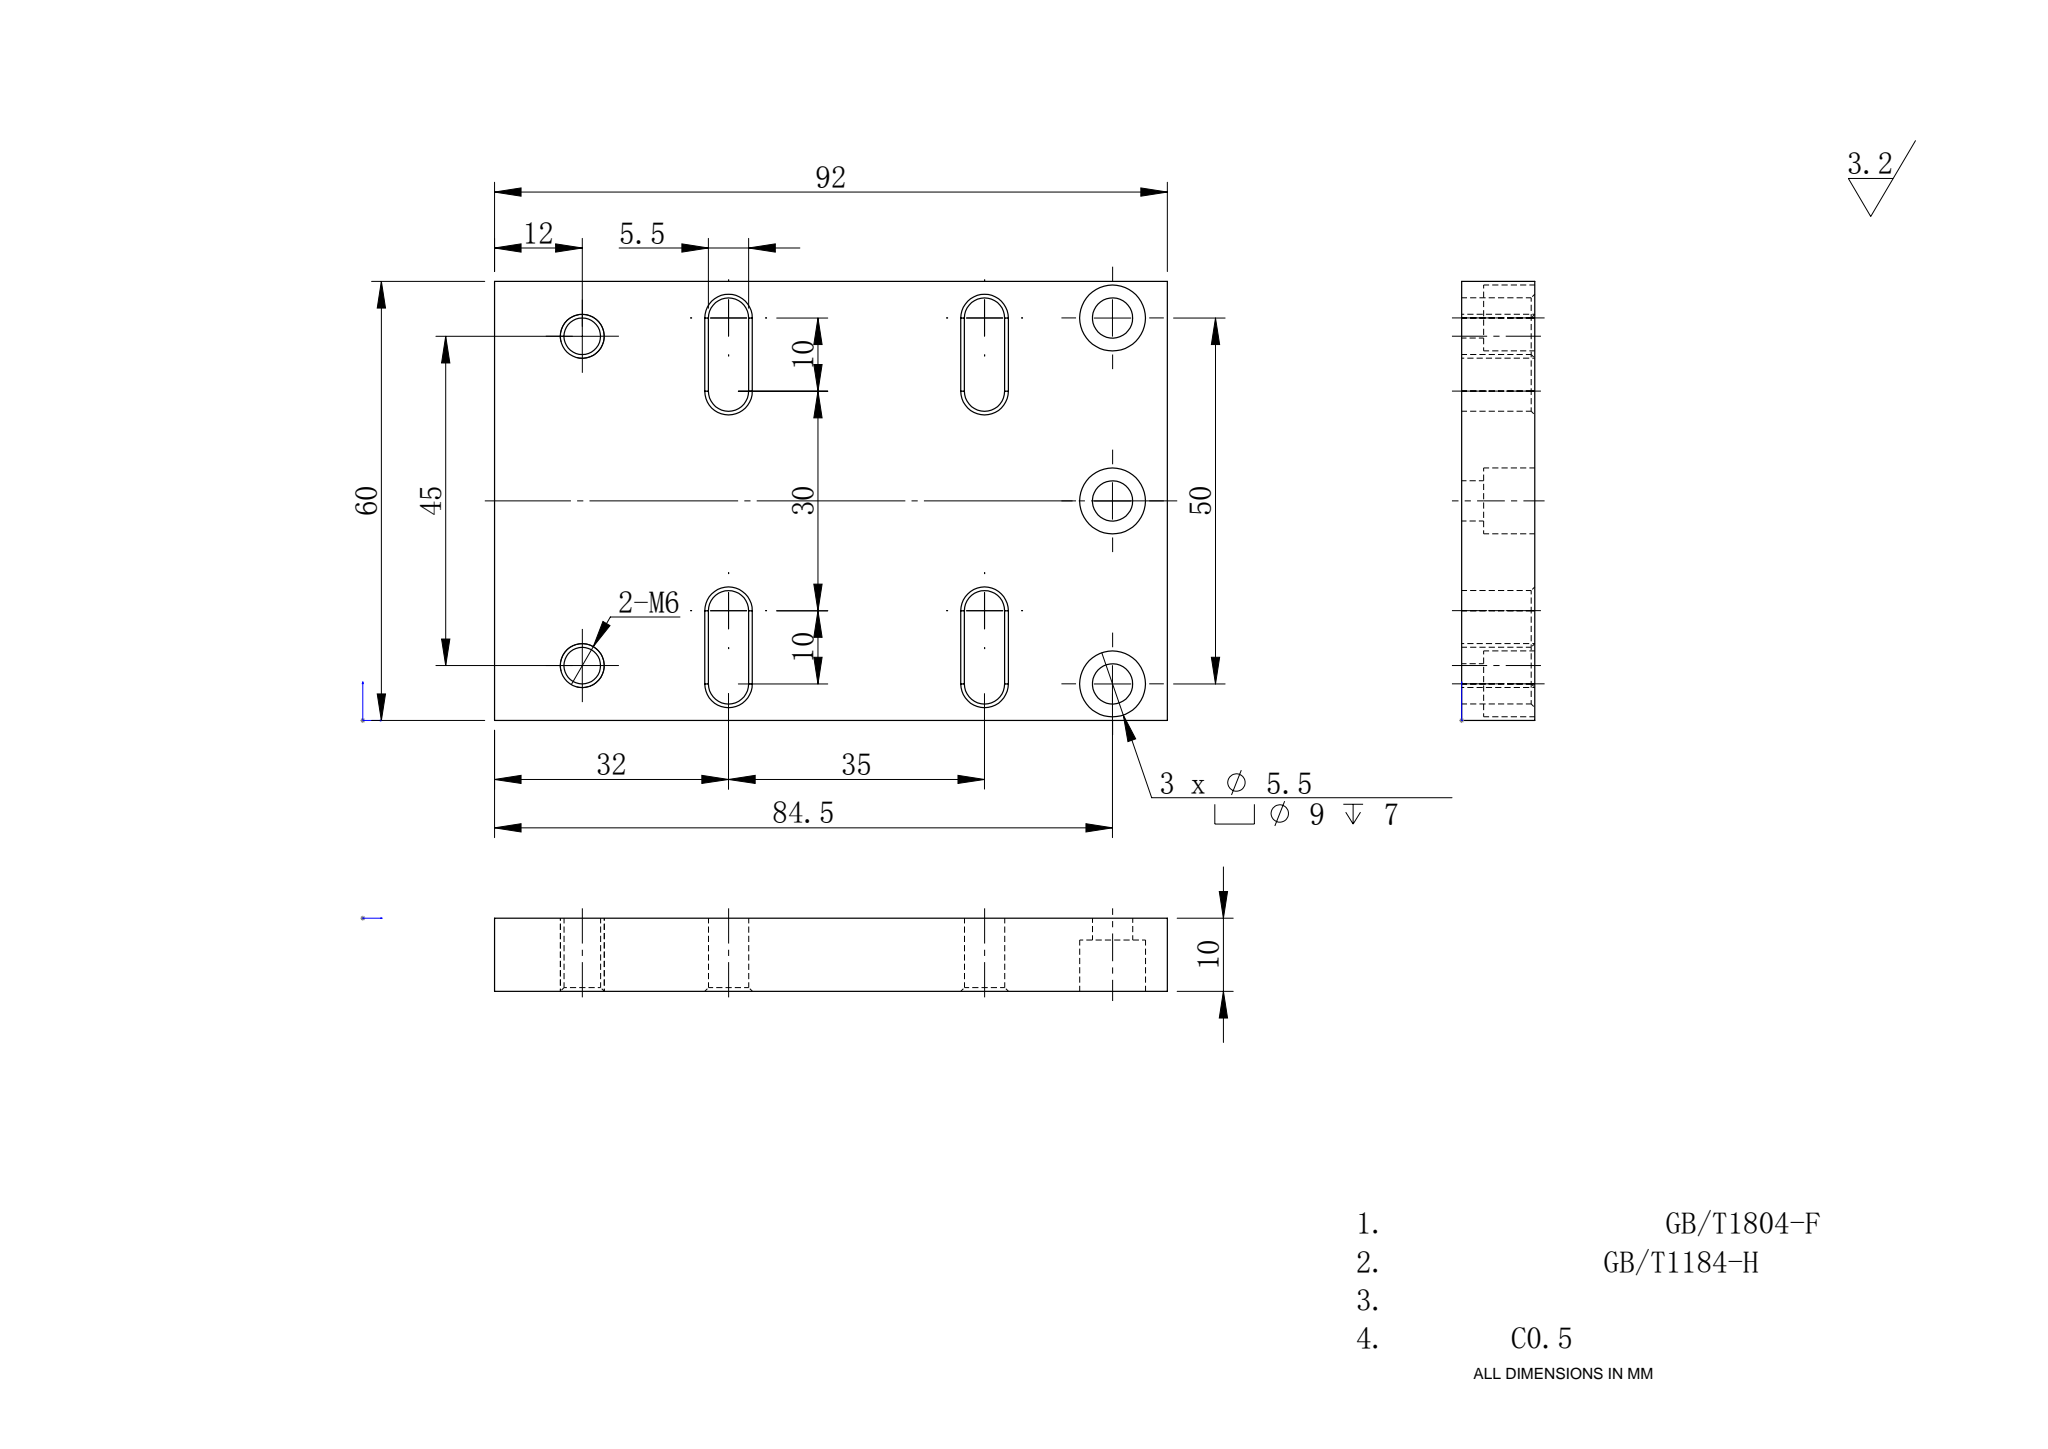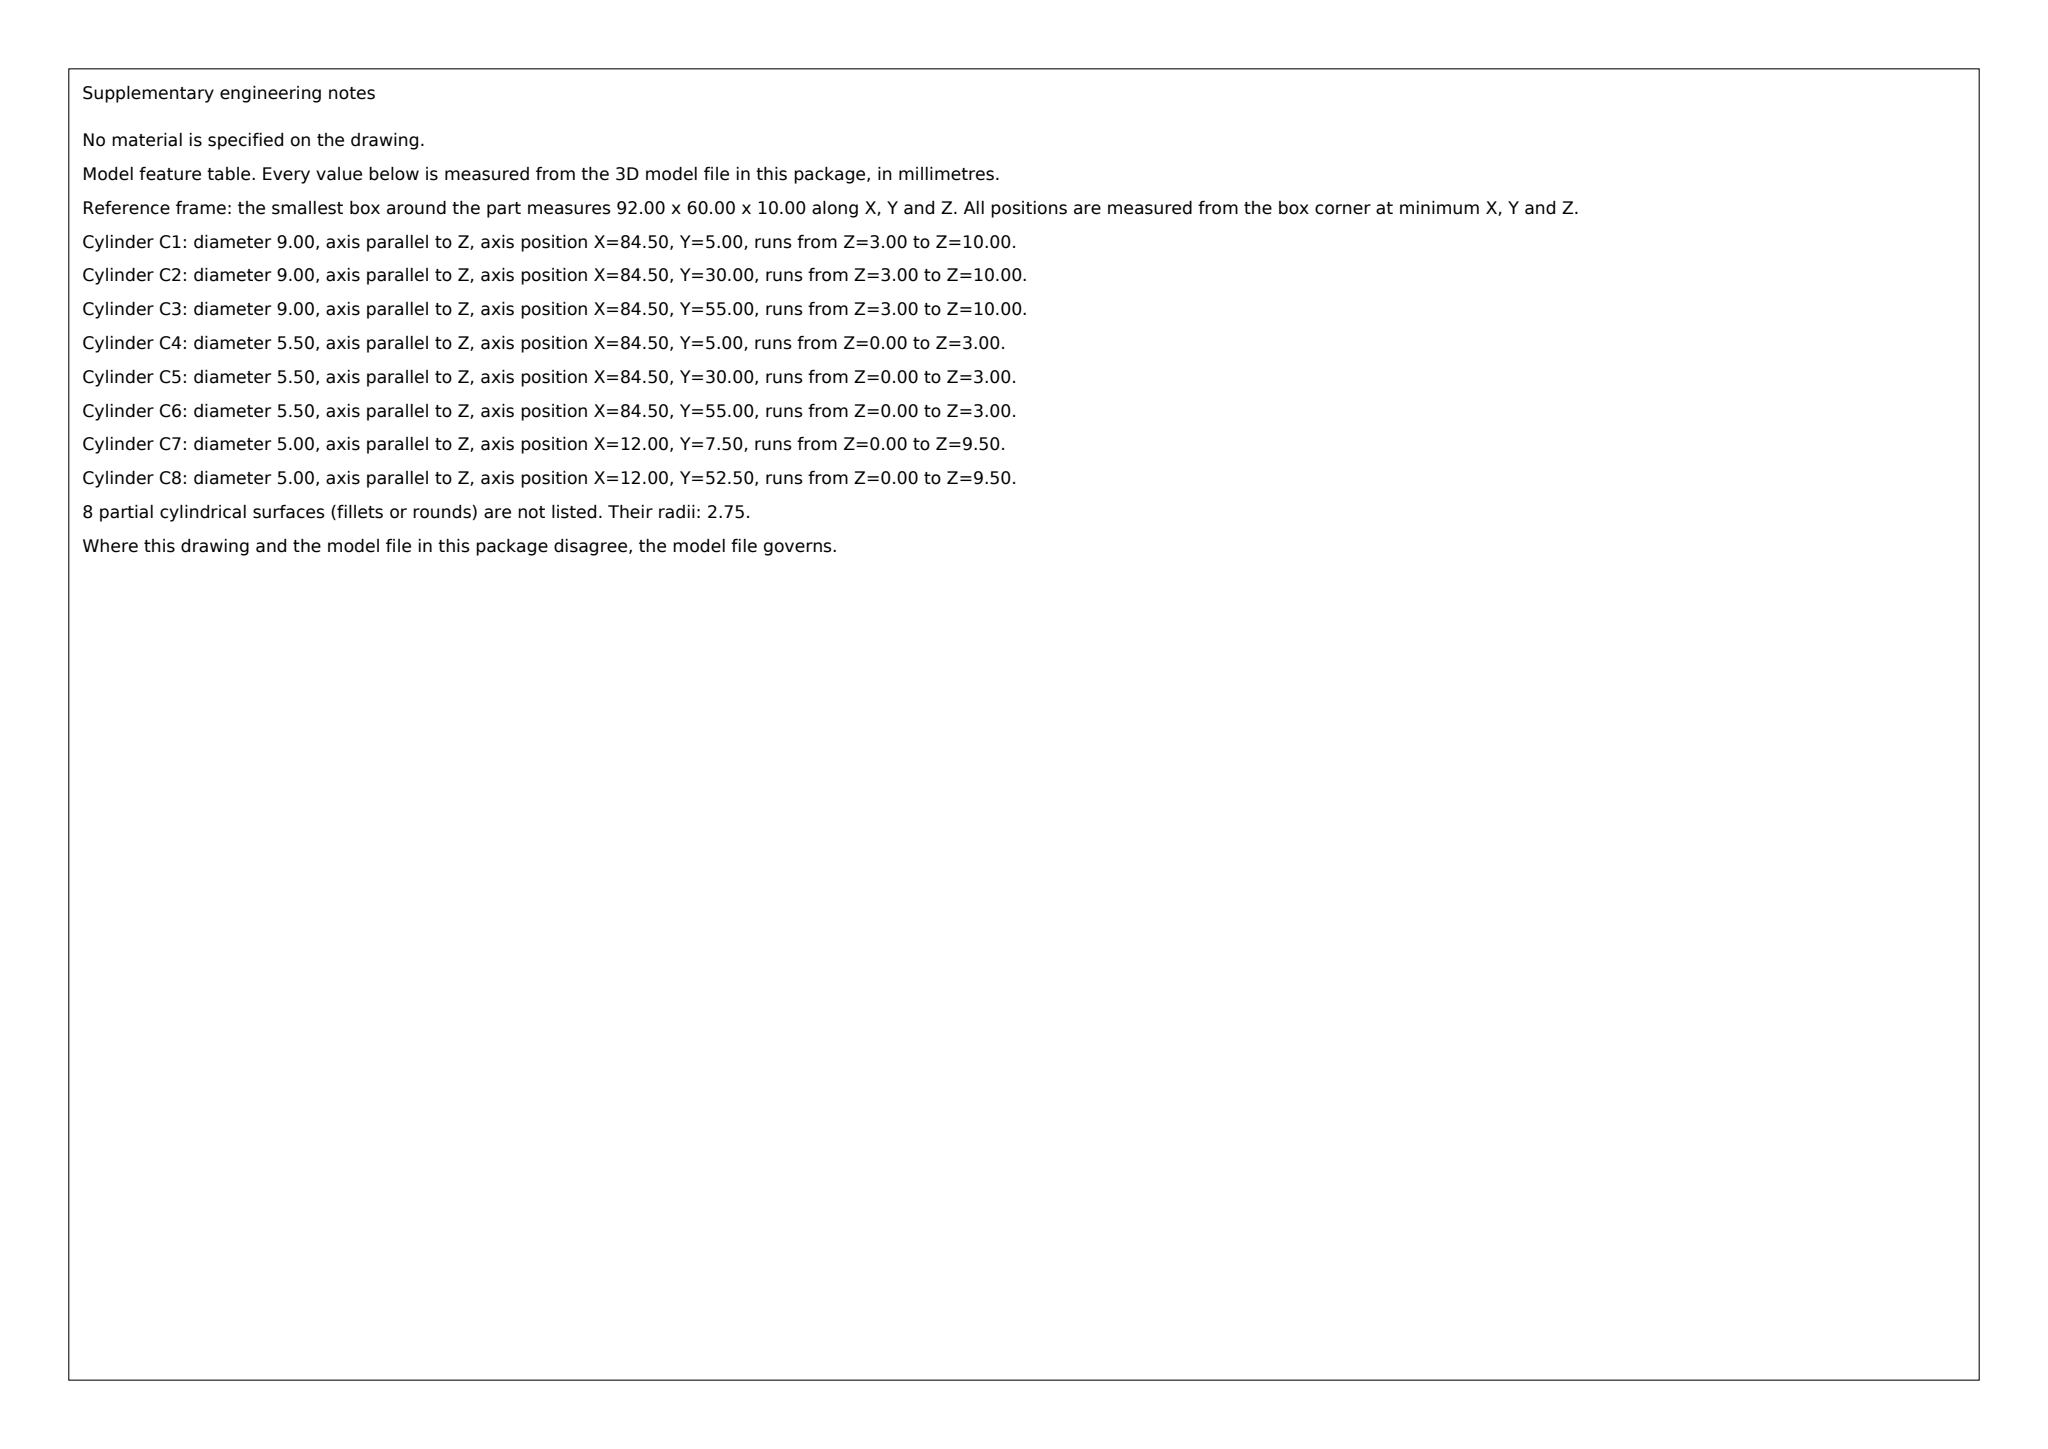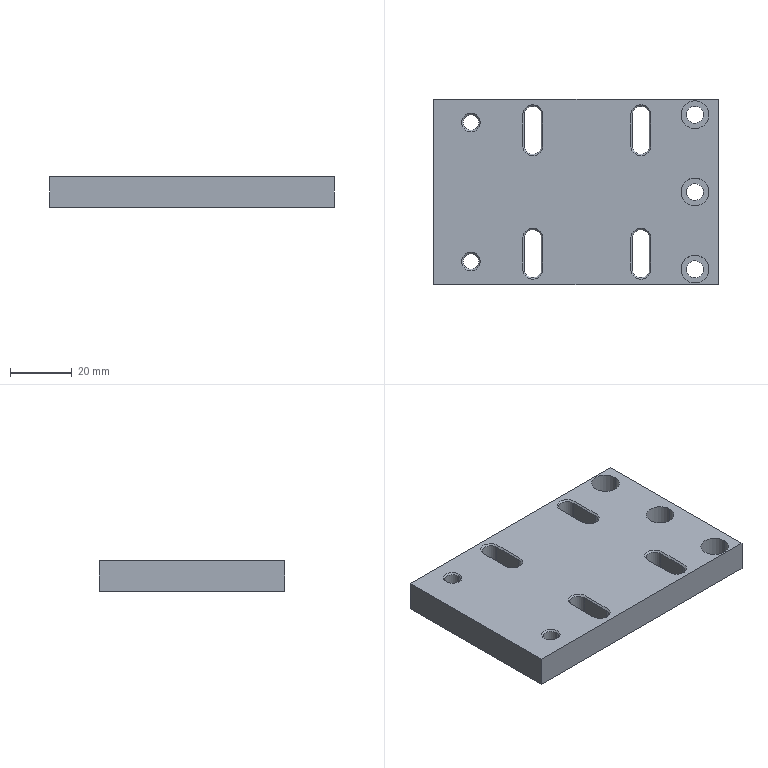Part | SolidWorks | mm | 1 solid | 61 faces | box 92 x 60 x 10 mm | volume 50084 mm3 | plane 25 | cylinder 24 | cone 12 | commonest cylinder face diameters 5.5 x14 9 x6 5 x4
build123d program:
from build123d import *

# Parameters (mm, degrees)
SKETCH1_W                                            = 110
SKETCH1_H                                            = 60
BOSS_EXTRUDE1_DEPTH                                  = 10
HOLE_SIZE_ACCORDING_TO_TYPE_1_OF_HEXAGON_D           = 5.5
HOLE_SIZE_ACCORDING_TO_TYPE_1_OF_HEXAGON_CBORE_D     = 9
HOLE_SIZE_ACCORDING_TO_TYPE_1_OF_HEXAGON_CBORE_DEPTH = 7
M6_TAPPED_HOLE1_D                                    = 5
CUT_EXTRUDE1_DEPTH                                   = 126.698
SKETCH7_W                                            = 18
SKETCH7_H                                            = 60
CUT_EXTRUDE2_DEPTH                                   = 126.698
CHAMFER1_SIZE                                        = 0.5
CHAMFER2_SIZE                                        = 0.5


with BuildPart() as part:
    # Sketch1 → Boss-Extrude1 (new body)
    with BuildSketch(Plane.XY):
        with Locations((55, 30)):
            Rectangle(SKETCH1_W, SKETCH1_H)
    extrude(amount=BOSS_EXTRUDE1_DEPTH)

    # Hole Size_According to_Type 1 of Hexagon (through all)
    with Locations(Plane(origin=(102.5, 55, 10), x_dir=(1, 0, 0), z_dir=(0, 0, 1))):
        with Locations((0, 0), (0, -25), (0, -50)):
            CounterBoreHole(HOLE_SIZE_ACCORDING_TO_TYPE_1_OF_HEXAGON_D / 2, HOLE_SIZE_ACCORDING_TO_TYPE_1_OF_HEXAGON_CBORE_D / 2, HOLE_SIZE_ACCORDING_TO_TYPE_1_OF_HEXAGON_CBORE_DEPTH)

    # M6 Tapped Hole1 (through all)
    with Locations(Plane(origin=(30, 52.5, 10), x_dir=(1, 0, 0), z_dir=(0, 0, 1))):
        with Locations((0, 0), (0, -45)):
            Hole(M6_TAPPED_HOLE1_D / 2)

    # Sketch6 → Cut-Extrude1 (cut, through all)
    with BuildSketch(Plane.XY.offset(10)):
        with BuildLine():
            Line((52.75, 55), (52.75, 45))
            ThreePointArc((52.75, 45), (50, 42.25), (47.25, 45))
            Line((47.25, 45), (47.25, 55))
            ThreePointArc((47.25, 55), (50, 57.75), (52.75, 55))
        make_face()
        with BuildLine():
            Line((87.75, 55), (87.75, 45))
            ThreePointArc((87.75, 45), (85, 42.25), (82.25, 45))
            Line((82.25, 45), (82.25, 55))
            ThreePointArc((82.25, 55), (85, 57.75), (87.75, 55))
        make_face()
        with BuildLine():
            Line((87.75, 15), (87.75, 5))
            ThreePointArc((87.75, 5), (85, 2.25), (82.25, 5))
            Line((82.25, 5), (82.25, 15))
            ThreePointArc((82.25, 15), (85, 17.75), (87.75, 15))
        make_face()
        with BuildLine():
            Line((52.75, 15), (52.75, 5))
            ThreePointArc((52.75, 5), (50, 2.25), (47.25, 5))
            Line((47.25, 5), (47.25, 15))
            ThreePointArc((47.25, 15), (50, 17.75), (52.75, 15))
        make_face()
    extrude(amount=-CUT_EXTRUDE1_DEPTH, mode=Mode.SUBTRACT)

    # Sketch7 → Cut-Extrude2 (cut, through all)
    with BuildSketch(Plane.XY.offset(10)):
        with Locations((9, 30)):
            Rectangle(SKETCH7_W, SKETCH7_H)
    extrude(amount=-CUT_EXTRUDE2_DEPTH, mode=Mode.SUBTRACT)

    # Chamfer1
    chamfer1_edges = [part.edges().sort_by_distance(p)[0] for p in [
        (50, 57.75, 10),
        (47.25, 50, 10),
        (50, 42.25, 10),
        (52.75, 50, 10),
        (85, 57.75, 10),
        (82.25, 50, 10),
        (85, 42.25, 10),
        (87.75, 50, 10),
        (85, 17.75, 10),
        (82.25, 10, 10),
        (85, 2.25, 10),
        (87.75, 10, 10),
        (50, 17.75, 10),
        (47.25, 10, 10),
        (50, 2.25, 10),
        (52.75, 10, 10),
    ]]
    chamfer(chamfer1_edges, length=CHAMFER1_SIZE)

    # Chamfer2
    chamfer2_edges = [part.edges().sort_by_distance(p)[0] for p in [
        (32.5, 7.5, 10),
        (32.5, 52.5, 10),
    ]]
    chamfer(chamfer2_edges, length=CHAMFER2_SIZE)


solid = part.part